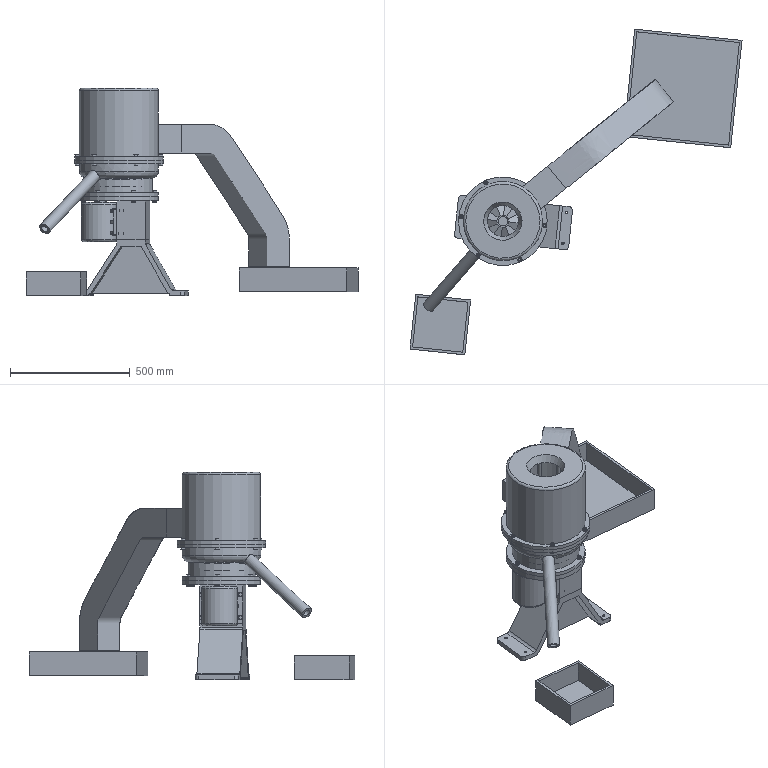Assembly | NX | mm | 44 component files | 44 solids | 1672 faces | box 1384.65 x 1358.4 x 865 mm | volume 31426566 mm3 | other 540 | plane 464 | cone 350 | cylinder 286 | torus 26 | spline 6 | commonest cylinder face diameters 96.75 x67 57.75 x41 11 x32 9.732 x24 8.5 x20 310 x14 17 x12 30 x11
Bill of materials:
unnamed part 1 | 1 |  | Hollow, stepped, round flanged sleeve. A thin outer flange has four through-holes, and a raised boss above it has four smaller holes.
unnamed part 2 | 1 |  | Hollow cylindrical boss with a thin base flange, plus a rectangular-section arm that runs out sideways and bends downward in two stages.
unnamed part 3 | 1 |  | Solid stepped cylindrical shaft or pin with several coaxial diameters, including one wider collar section.
unnamed part 4 | 1 |  | Open-top square box or tray with thin, uniform walls, a flat floor and relatively tall sides.
GB-T5782-2000,M10x45 | 6 |  | Hexagon Head Bolt, GB-T 5782-2000,M10x45
GB-T6170_F-2000,M10x1.5 | 12 |  | Hexagonal nut-shaped block with a plain central through-bore and chamfered corners on both faces.
unnamed part 5 | 1 |  | Round disc with a cylindrical edge band and a shallow cone-shaped top. The top is faceted in a six-pointed star pattern and has a small central hub with a through-hole.
GB-T5782-2000,M10x25 | 3 |  | Hexagon Head Bolt, GB-T 5782-2000,M10x25
GB-T5782-2000,M10x20 | 1 |  | Hexagon Head Bolt, GB-T 5782-2000,M10x20
unnamed part 6 | 1 |  | Bent-plate, hat-shaped bracket: a raised flat top joined by two sloping legs to two outward-facing feet, with a triangular side web on one side.
GB-T5781-2000,M10x40 | 6 |  | Hex-headed bolt-like solid: a short hexagonal prism head with a long, plain cylindrical shank coaxial with it. The shank is several head-heights long and has a chamfered free end.
GB-T5781-2000,M10x25 | 4 |  | Hex-headed bolt-like solid: a hexagonal prism head with a coaxial plain cylindrical shank. The shank is shorter relative to the head than in the other part. The top of the head is chamfered and the shank tip is chamfered.
unnamed part 7 | 1 |  | Short cylindrical, bowl-like housing with a top and bottom flange, a floor with a central hole, and a hollow tube coming out of the side at an angle.
unnamed part 8 | 1 |  | Rounded cylindrical body with a coaxial stepped shaft sticking out of one end. A rectangular mounting plate with four corner holes stands off one side on a triangular support.
unnamed part 9 | 1 |  | Spur-gear-shaped disc with straight teeth all around the rim and a central bore with one keyway.
unnamed part 10 | 1 |  | Shallow, open-top square tray with thin walls and a flat floor.
unnamed part 11 | 1 |  | Round flat plate with a rectangular hollow box underneath, set off-centre. The plate has a large round hole, a rectangular opening into the box, and several small holes.
unnamed part 12 | 1 |  | Flat disc-shaped spur gear with many fine straight teeth around the outside and a plain round hole through the center. Both faces are flat, with no hub, web recess or spokes.
Mates:
1. touch align | conn_support 1 face | bracket 1 face
2. touch align | conn_support 1 face | bracket 1 face
3. touch align | conn_support 1 face | bracket 1 face
4. touch align | motor 1 face | conn_support 1 face
5. touch align | motor 1 face | conn_support 1 face
6. touch align | motor 1 face | conn_support 1 face
7. touch align | gearbox 1 face | conn_support 1 face
8. touch align | gearbox 1 face | conn_support 1 face
9. touch align | gearbox 1 face | conn_support 1 face
10. touch align | storage_bin 1 face | gearbox 1 face
11. touch align | storage_bin 1 face | gearbox 1 face
12. touch align | storage_bin 1 face | gearbox 1 face
13. touch align | roller 1 face | gearbox 1 face
14. distance | roller 1 face | gearbox 1 face
15. parallel | storage_box 1 face | bracket 1 face
16. distance | storage_box 1 face | bracket 1 face
17. distance | storage_box 1 face | bracket 1 face
18. touch align | square_box 1 face | bracket 1 face
19. distance | square_box 1 face | bracket 1 face
20. distance | square_box 1 face | bracket 1 face
21. touch align | flange 1 face | gearbox 1 face
22. touch align | flange 1 face | roller 1 face
23. touch align | driven_gear 1 face | gearbox 1 face
24. fix | bracket 1 component
25. touch align | drive_gear 1 face | motor 1 face
26. touch align | motor 1 face | drive_gear 1 face
27. touch align | drive_gear 1 face | motor 1 edge
28. touch align | GB-T5782-2000_M10x25 3 face | motor 1 face
29. touch align | GB-T5782-2000_M10x25 3 face | motor 1 face
30. touch align | GB-T6170_F-2000_M10x1_5 12 face | gearbox 1 face
31. fix | assembly component
32. bond | GB-T6170_F-2000_M10x1_5 12 component | assembly component
33. bond | GB-T5782-2000_M10x45 6 component | assembly component
34. bond | GB-T6170_F-2000_M10x1_5 11 component | assembly component
35. bond | GB-T5782-2000_M10x45 5 component | assembly component
36. bond | GB-T6170_F-2000_M10x1_5 10 component | assembly component
37. bond | GB-T5782-2000_M10x45 4 component | assembly component
38. bond | GB-T6170_F-2000_M10x1_5 9 component | assembly component
39. bond | GB-T5782-2000_M10x45 3 component | assembly component
40. circular | assembly datumaxis | assembly cartesiancoordinatesystem | assembly cartesiancoordinatesystem | assembly cartesiancoordinatesystem | assembly cartesiancoordinatesystem | assembly cartesiancoordinatesystem | assembly cartesiancoordinatesystem
41. circular | assembly datumaxis | assembly cartesiancoordinatesystem | assembly cartesiancoordinatesystem | assembly cartesiancoordinatesystem | assembly cartesiancoordinatesystem | assembly cartesiancoordinatesystem | assembly cartesiancoordinatesystem
42. bond | GB-T6170_F-2000_M10x1_5 8 component | assembly component
43. bond | GB-T5782-2000_M10x45 2 component | assembly component
44. bond | GB-T6170_F-2000_M10x1_5 7 component | assembly component
45. bond | GB-T5782-2000_M10x45 1 component | assembly component
46. touch align | GB-T5782-2000_M10x25 2 face | motor 1 face
47. touch align | GB-T5782-2000_M10x25 1 face | motor 1 face
48. touch align | GB-T5782-2000_M10x20 1 face | motor 1 face
49. touch align | GB-T6170_F-2000_M10x1_5 6 face | storage_bin 1 face
50. fix | assembly component
51. bond | GB-T6170_F-2000_M10x1_5 6 component | assembly component
52. bond | GB-T5781-2000_M10x40 6 component | assembly component
53. bond | GB-T6170_F-2000_M10x1_5 5 component | assembly component
54. bond | GB-T5781-2000_M10x40 5 component | assembly component
55. bond | GB-T6170_F-2000_M10x1_5 4 component | assembly component
56. bond | GB-T5781-2000_M10x40 4 component | assembly component
57. bond | GB-T6170_F-2000_M10x1_5 3 component | assembly component
58. bond | GB-T5781-2000_M10x40 3 component | assembly component
59. bond | GB-T6170_F-2000_M10x1_5 2 component | assembly component
60. bond | GB-T5781-2000_M10x40 2 component | assembly component
61. bond | GB-T6170_F-2000_M10x1_5 1 component | assembly component
62. bond | GB-T5781-2000_M10x40 1 component | assembly component
63. circular | assembly datumaxis | assembly cartesiancoordinatesystem | assembly cartesiancoordinatesystem | assembly cartesiancoordinatesystem | assembly cartesiancoordinatesystem | assembly cartesiancoordinatesystem | assembly cartesiancoordinatesystem
64. circular | assembly datumaxis | assembly cartesiancoordinatesystem | assembly cartesiancoordinatesystem | assembly cartesiancoordinatesystem | assembly cartesiancoordinatesystem | assembly cartesiancoordinatesystem | assembly cartesiancoordinatesystem